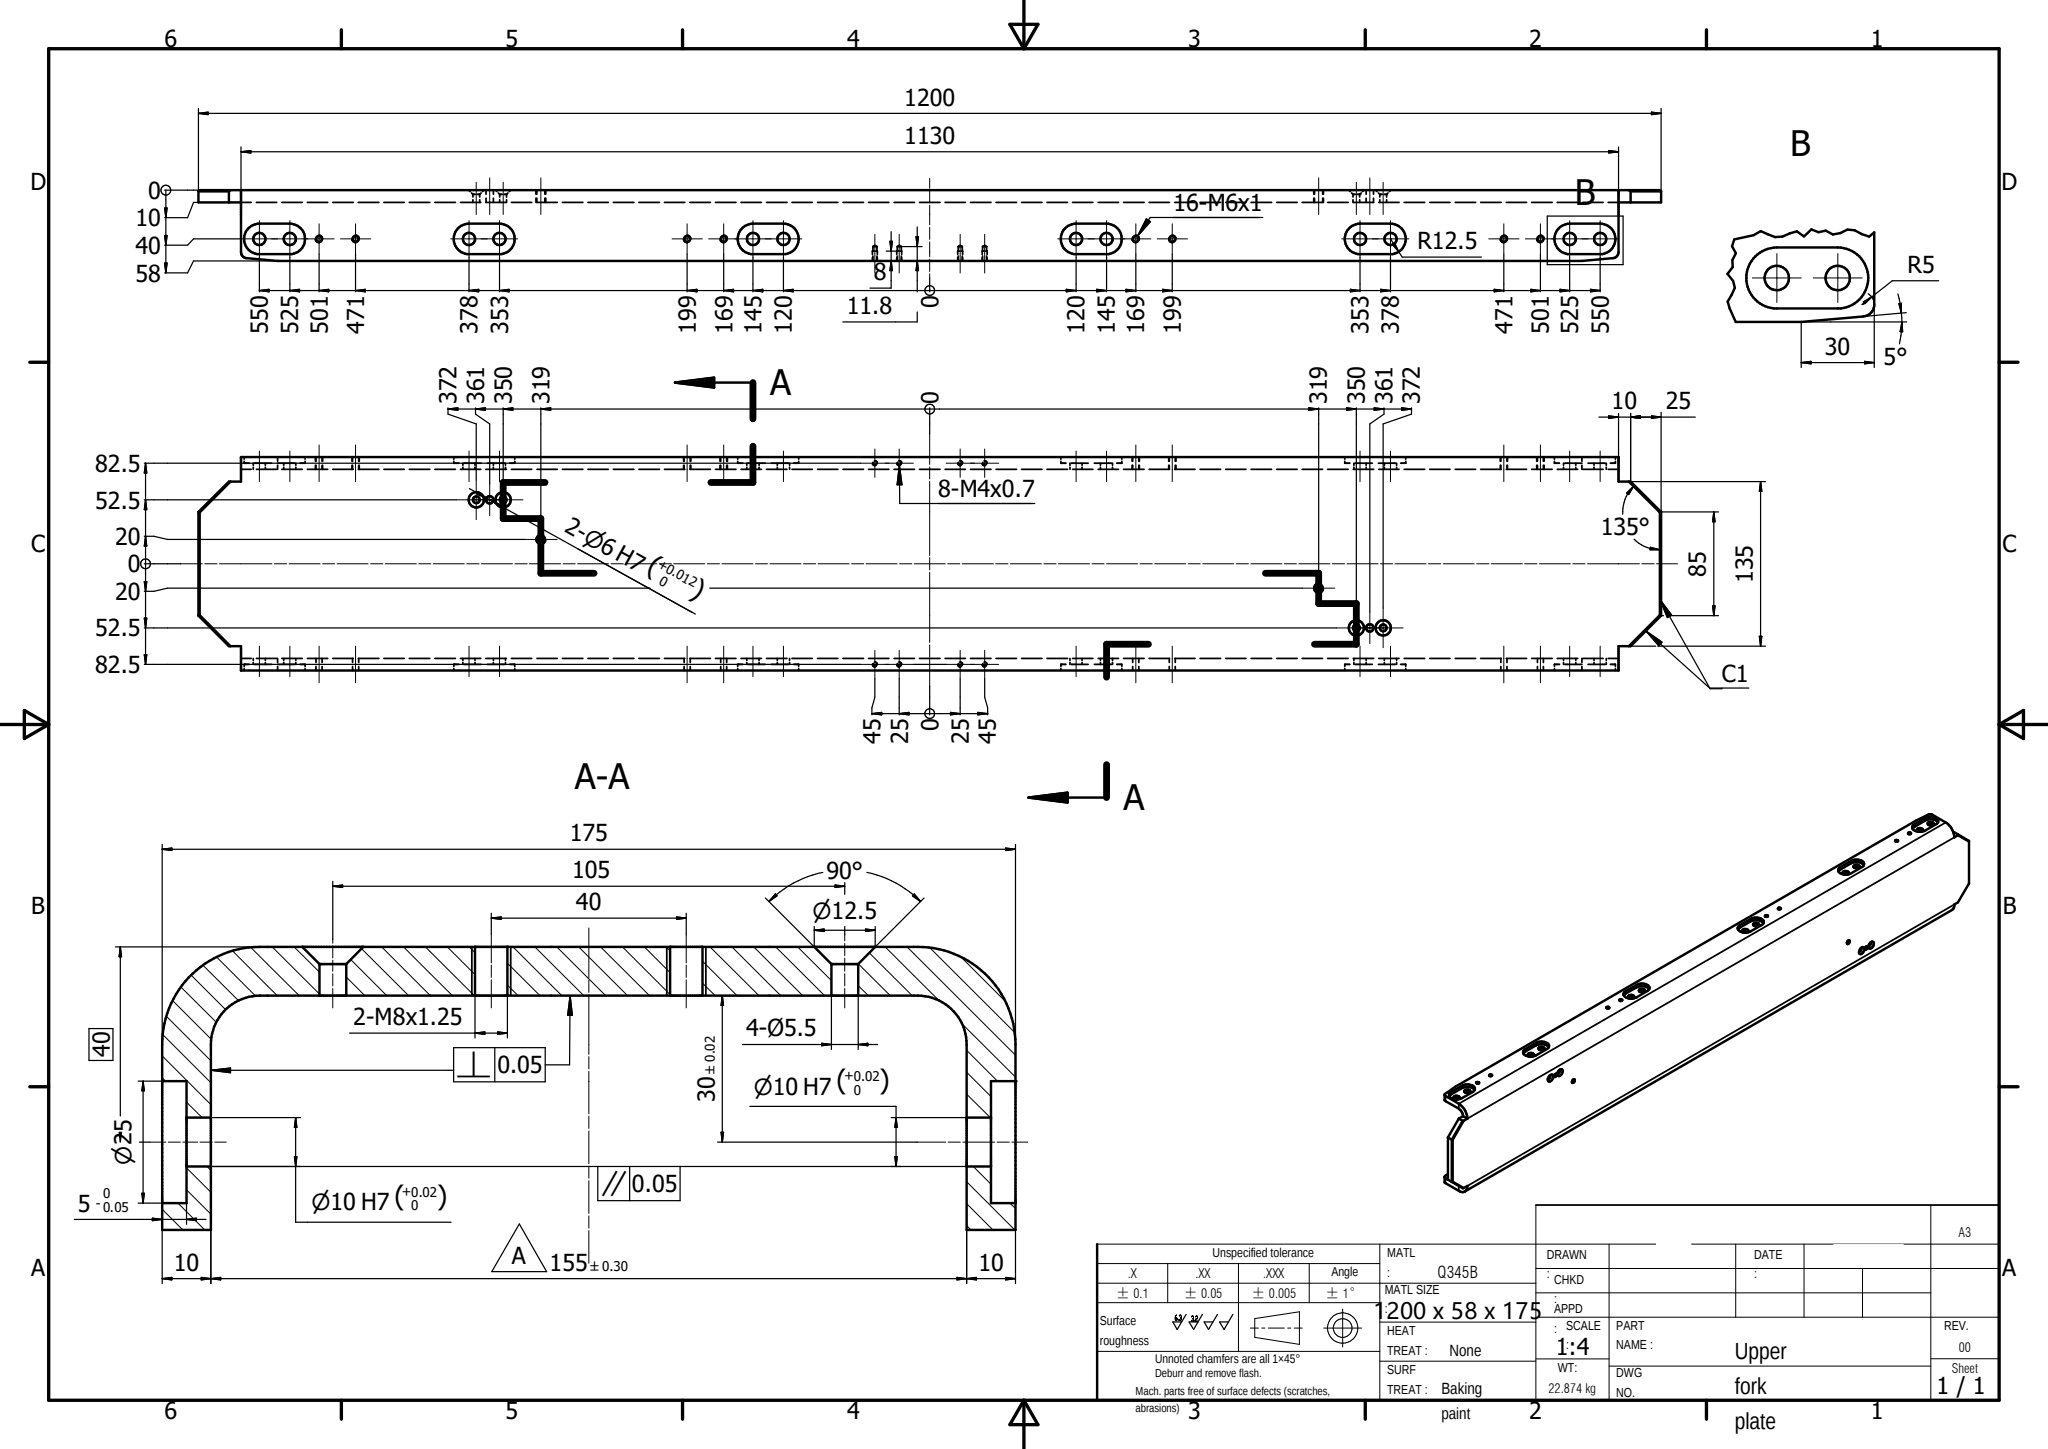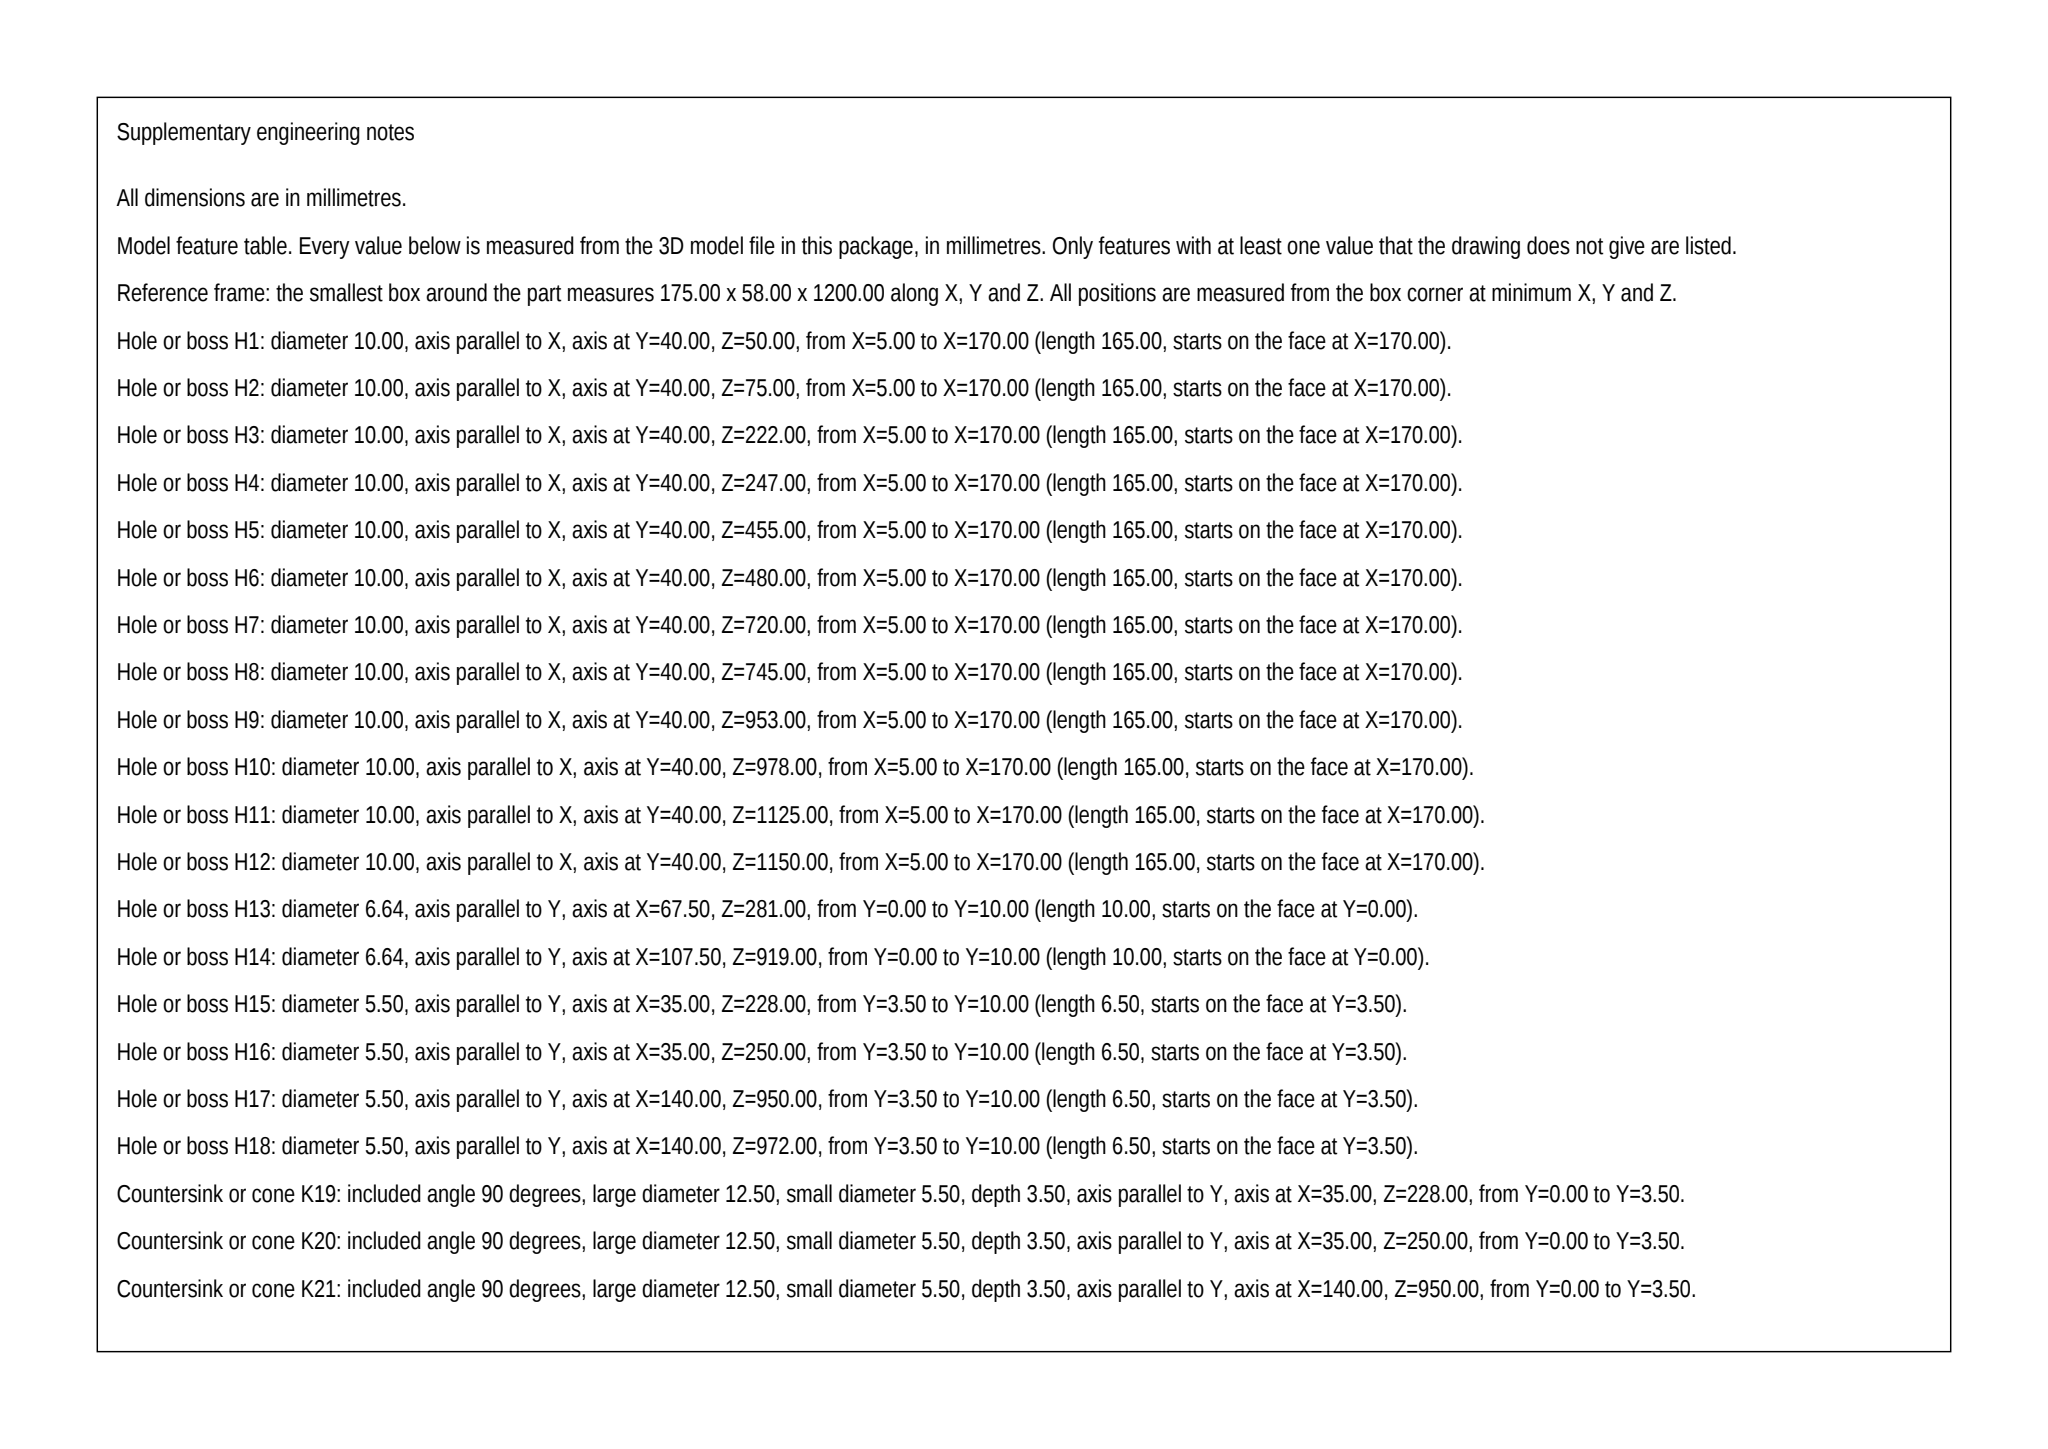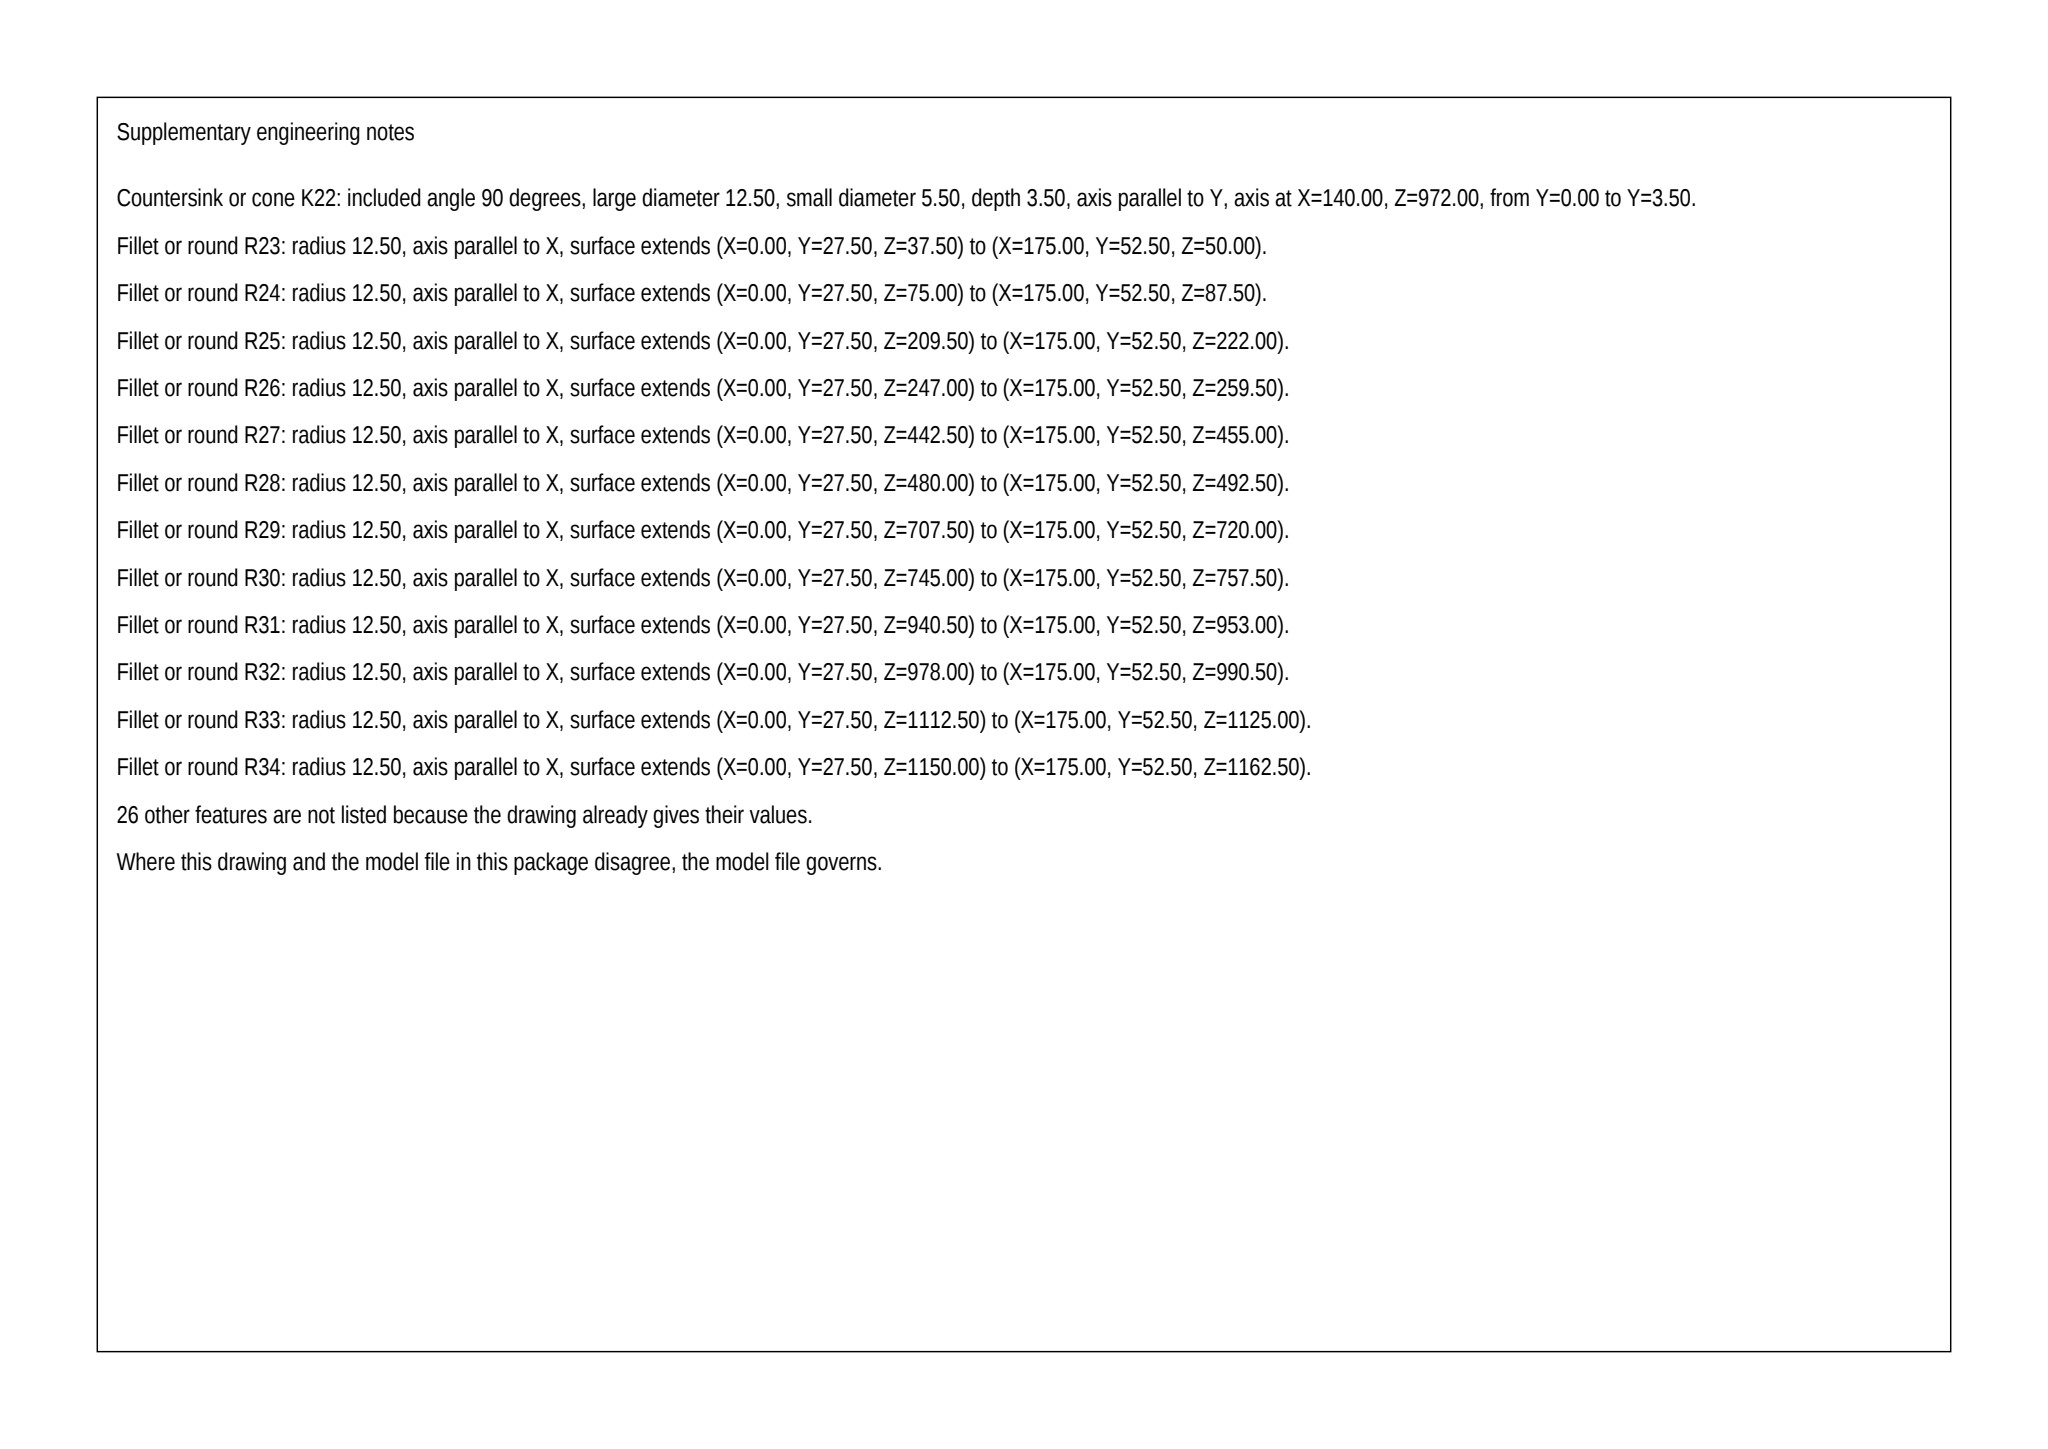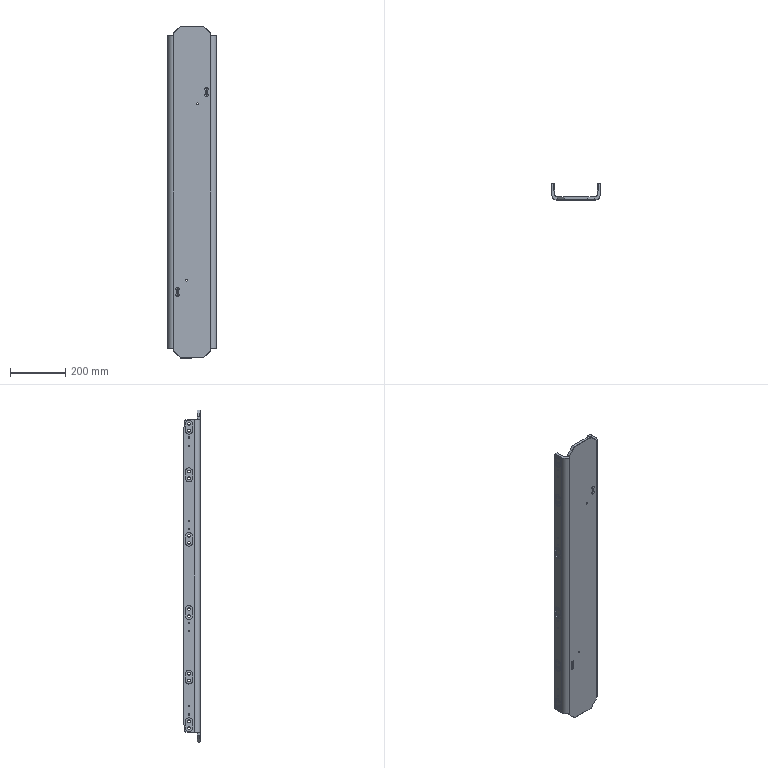Part | SolidWorks | mm | 1 solid | 248 faces | box 175 x 58 x 1200 mm | volume 2913866 mm3 | cylinder 156 | plane 68 | cone 24 | commonest cylinder face diameters 10 x52 25 x36 4.917 x32 3.242 x16 5.5 x8 6 x4 6.647 x4 20 x2
Drawing notes:
SECT A-A BEND RADII: R10 INSIDE, R20 OUTSIDE, TYP 2 CORNERS | from the solid: cylinders dia 20.0 & 40.0 axis z at (x20,y20) and (x155,y20), length 1130 = inner R10 / outer R20 web-to-leg bends
4-Ø10 THRU LEG WALLS: 40 FROM EA END, CL 50.79 FROM 0 DATUM | from the solid: cyl dia 10.0 axis x, pos y=50.79, z=40 and z=1160, len 10, count 2 each (both legs); bbox length 1200 -> 40 from each end